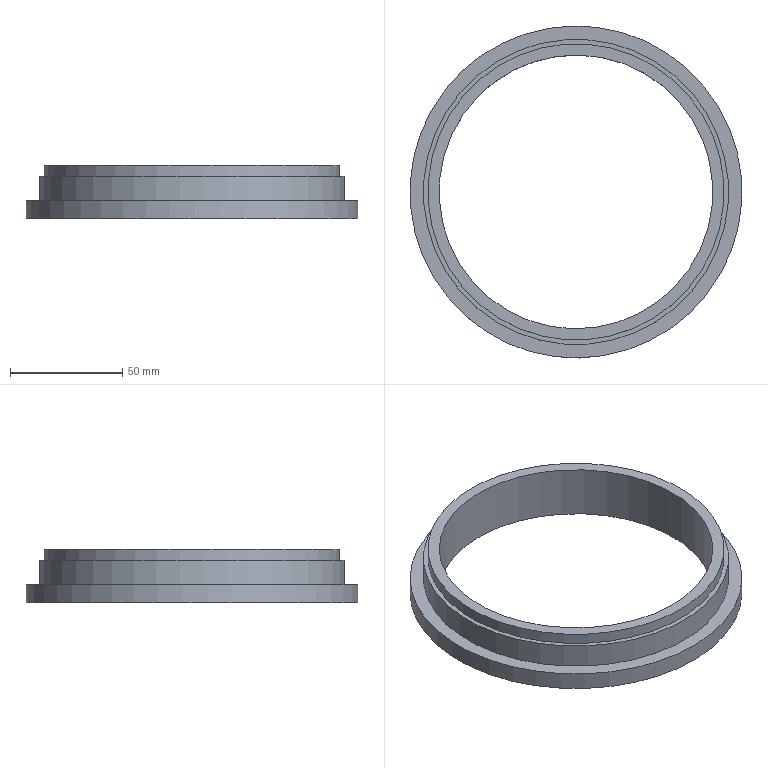Component | NX | CH3404-8 | 1 solid | 8 faces | box 148 x 148 x 24 mm | volume 85288 mm3 | cylinder 4 | plane 4 | commonest cylinder face diameters 122 x1 132 x1 136 x1 148 x1
STEP:
#1=CARTESIAN_POINT('',(0.,0.,0.));
#2=DIRECTION('',(0.,0.,1.));
#3=DIRECTION('',(1.,0.,0.));
#4=AXIS2_PLACEMENT_3D('',#1,#2,#3);
#5=CARTESIAN_POINT('',(56.878,23.472,-1551.3));
#6=VERTEX_POINT('',#5);
#7=CARTESIAN_POINT('',(0.5308,0.1057,-1551.3));
#8=DIRECTION('',(0.,0.,1.));
#9=DIRECTION('',(0.9237,0.383,0.));
#10=AXIS2_PLACEMENT_3D('',#7,#8,#9);
#11=CIRCLE('',#10,61.);
#12=CARTESIAN_POINT('',(0.5308,0.1057,-1551.3));
#13=DIRECTION('',(0.,0.,1.));
#14=DIRECTION('',(0.9237,0.383,0.));
#15=AXIS2_PLACEMENT_3D('',#12,#13,#14);
#16=CYLINDRICAL_SURFACE('',#15,61.);
#17=CARTESIAN_POINT('',(0.,0.));
#18=DIRECTION('',(1.,0.));
#19=VECTOR('',#18,1.);
#20=LINE('',#17,#19);
#21=(GEOMETRIC_REPRESENTATION_CONTEXT(2)PARAMETRIC_REPRESENTATION_CONTEXT()REPRESENTATION_CONTEXT('',''));
#22=DEFINITIONAL_REPRESENTATION('',(#20),#21);
#23=PCURVE('',#16,#22);
#24=CARTESIAN_POINT('',(-22.835,56.453,-1551.3));
#25=DIRECTION('',(0.,0.,1.));
#26=DIRECTION('',(0.9237,0.383,0.));
#27=AXIS2_PLACEMENT_3D('',#24,#25,#26);
#28=PLANE('',#27);
#29=CARTESIAN_POINT('',(-0.,-61.));
#30=DIRECTION('',(1.,0.));
#31=AXIS2_PLACEMENT_2D('',#29,#30);
#32=CIRCLE('',#31,61.);
#33=(GEOMETRIC_REPRESENTATION_CONTEXT(2)PARAMETRIC_REPRESENTATION_CONTEXT()REPRESENTATION_CONTEXT('',''));
#34=DEFINITIONAL_REPRESENTATION('',(#32),#33);
#35=PCURVE('',#28,#34);
#36=SURFACE_CURVE('',#11,(#23,#35),.PCURVE_S1.);
#37=EDGE_CURVE('',#6,#6,#36,.T.);
#38=ORIENTED_EDGE('',*,*,#37,.F.);
#39=CARTESIAN_POINT('',(56.878,23.472,-1575.3));
#40=VERTEX_POINT('',#39);
#41=CARTESIAN_POINT('',(56.878,23.472,-1575.3));
#42=CARTESIAN_POINT('',(56.878,23.472,-1551.3));
#43=B_SPLINE_CURVE_WITH_KNOTS('',1,(#41,#42),.UNSPECIFIED.,.F.,.F.,(2,2),(-24.,0.),.PIECEWISE_BEZIER_KNOTS.);
#44=CARTESIAN_POINT('',(0.,0.));
#45=DIRECTION('',(0.,1.));
#46=VECTOR('',#45,1.);
#47=LINE('',#44,#46);
#48=(GEOMETRIC_REPRESENTATION_CONTEXT(2)PARAMETRIC_REPRESENTATION_CONTEXT()REPRESENTATION_CONTEXT('',''));
#49=DEFINITIONAL_REPRESENTATION('',(#47),#48);
#50=PCURVE('',#16,#49);
#51=CARTESIAN_POINT('',(6.283,0.));
#52=DIRECTION('',(0.,1.));
#53=VECTOR('',#52,1.);
#54=LINE('',#51,#53);
#55=(GEOMETRIC_REPRESENTATION_CONTEXT(2)PARAMETRIC_REPRESENTATION_CONTEXT()REPRESENTATION_CONTEXT('',''));
#56=DEFINITIONAL_REPRESENTATION('',(#54),#55);
#57=PCURVE('',#16,#56);
#58=SEAM_CURVE('',#43,(#50,#57),.PCURVE_S1.);
#59=EDGE_CURVE('',#40,#6,#58,.T.);
#60=ORIENTED_EDGE('',*,*,#59,.F.);
#61=CARTESIAN_POINT('',(0.5308,0.1057,-1575.3));
#62=DIRECTION('',(0.,0.,1.));
#63=DIRECTION('',(0.9237,0.383,0.));
#64=AXIS2_PLACEMENT_3D('',#61,#62,#63);
#65=CIRCLE('',#64,61.);
#66=CARTESIAN_POINT('',(0.,-24.));
#67=DIRECTION('',(1.,0.));
#68=VECTOR('',#67,1.);
#69=LINE('',#66,#68);
#70=(GEOMETRIC_REPRESENTATION_CONTEXT(2)PARAMETRIC_REPRESENTATION_CONTEXT()REPRESENTATION_CONTEXT('',''));
#71=DEFINITIONAL_REPRESENTATION('',(#69),#70);
#72=PCURVE('',#16,#71);
#73=CARTESIAN_POINT('',(-27.815,68.462,-1575.3));
#74=DIRECTION('',(0.,0.,-1.));
#75=DIRECTION('',(-0.9237,-0.383,0.));
#76=AXIS2_PLACEMENT_3D('',#73,#74,#75);
#77=PLANE('',#76);
#78=CARTESIAN_POINT('',(-61.,-74.));
#79=CARTESIAN_POINT('',(-61.,31.655));
#80=CARTESIAN_POINT('',(30.5,-21.172));
#81=CARTESIAN_POINT('',(122.,-74.));
#82=CARTESIAN_POINT('',(30.5,-126.828));
#83=CARTESIAN_POINT('',(-61.,-179.655));
#84=CARTESIAN_POINT('',(-61.,-74.));
#85=(BOUNDED_CURVE()B_SPLINE_CURVE(2,(#78,#79,#80,#81,#82,#83,#84),.UNSPECIFIED.,.T.,.F.)B_SPLINE_CURVE_WITH_KNOTS((1,2,2,2,2,1),(-2.094,0.,2.094,4.189,6.283,8.378),.UNSPECIFIED.)CURVE()GEOMETRIC_REPRESENTATION_ITEM()RATIONAL_B_SPLINE_CURVE((1.,0.5,1.,0.5,1.,0.5,1.))REPRESENTATION_ITEM(''));
#86=(GEOMETRIC_REPRESENTATION_CONTEXT(2)PARAMETRIC_REPRESENTATION_CONTEXT()REPRESENTATION_CONTEXT('',''));
#87=DEFINITIONAL_REPRESENTATION('',(#85),#86);
#88=PCURVE('',#77,#87);
#89=SURFACE_CURVE('',#65,(#72,#88),.PCURVE_S1.);
#90=EDGE_CURVE('',#40,#40,#89,.T.);
#91=ORIENTED_EDGE('',*,*,#90,.T.);
#92=ORIENTED_EDGE('',*,*,#59,.T.);
#93=EDGE_LOOP('',(#38,#60,#91,#92));
#94=FACE_BOUND('',#93,.F.);
#95=ADVANCED_FACE('',(#94),#16,.F.);
#96=CARTESIAN_POINT('',(61.497,25.387,-1551.3));
#97=VERTEX_POINT('',#96);
#98=CARTESIAN_POINT('',(0.5308,0.1057,-1551.3));
#99=DIRECTION('',(0.,0.,1.));
#100=DIRECTION('',(0.9237,0.383,0.));
#101=AXIS2_PLACEMENT_3D('',#98,#99,#100);
#102=CIRCLE('',#101,66.);
#103=CARTESIAN_POINT('',(-0.,-61.));
#104=DIRECTION('',(1.,0.));
#105=AXIS2_PLACEMENT_2D('',#103,#104);
#106=CIRCLE('',#105,66.);
#107=(GEOMETRIC_REPRESENTATION_CONTEXT(2)PARAMETRIC_REPRESENTATION_CONTEXT()REPRESENTATION_CONTEXT('',''));
#108=DEFINITIONAL_REPRESENTATION('',(#106),#107);
#109=PCURVE('',#28,#108);
#110=CARTESIAN_POINT('',(0.5308,0.1057,-1551.3));
#111=DIRECTION('',(0.,0.,1.));
#112=DIRECTION('',(0.9237,0.383,0.));
#113=AXIS2_PLACEMENT_3D('',#110,#111,#112);
#114=CYLINDRICAL_SURFACE('',#113,66.);
#115=CARTESIAN_POINT('',(0.,0.));
#116=DIRECTION('',(1.,0.));
#117=VECTOR('',#116,1.);
#118=LINE('',#115,#117);
#119=(GEOMETRIC_REPRESENTATION_CONTEXT(2)PARAMETRIC_REPRESENTATION_CONTEXT()REPRESENTATION_CONTEXT('',''));
#120=DEFINITIONAL_REPRESENTATION('',(#118),#119);
#121=PCURVE('',#114,#120);
#122=SURFACE_CURVE('',#102,(#109,#121),.PCURVE_S1.);
#123=EDGE_CURVE('',#97,#97,#122,.T.);
#124=ORIENTED_EDGE('',*,*,#123,.T.);
#125=EDGE_LOOP('',(#124));
#126=FACE_BOUND('',#125,.T.);
#127=ORIENTED_EDGE('',*,*,#37,.F.);
#128=EDGE_LOOP('',(#127));
#129=FACE_BOUND('',#128,.T.);
#130=ADVANCED_FACE('',(#126,#129),#28,.T.);
#131=CARTESIAN_POINT('',(61.497,25.387,-1556.3));
#132=VERTEX_POINT('',#131);
#133=CARTESIAN_POINT('',(0.5308,0.1057,-1556.3));
#134=DIRECTION('',(0.,0.,1.));
#135=DIRECTION('',(0.9237,0.383,0.));
#136=AXIS2_PLACEMENT_3D('',#133,#134,#135);
#137=CIRCLE('',#136,66.);
#138=CARTESIAN_POINT('',(0.,-5.));
#139=DIRECTION('',(1.,0.));
#140=VECTOR('',#139,1.);
#141=LINE('',#138,#140);
#142=(GEOMETRIC_REPRESENTATION_CONTEXT(2)PARAMETRIC_REPRESENTATION_CONTEXT()REPRESENTATION_CONTEXT('',''));
#143=DEFINITIONAL_REPRESENTATION('',(#141),#142);
#144=PCURVE('',#114,#143);
#145=CARTESIAN_POINT('',(-24.75,61.072,-1556.3));
#146=DIRECTION('',(0.,0.,1.));
#147=DIRECTION('',(0.9237,0.383,0.));
#148=AXIS2_PLACEMENT_3D('',#145,#146,#147);
#149=PLANE('',#148);
#150=CARTESIAN_POINT('',(-0.,-66.));
#151=DIRECTION('',(1.,0.));
#152=AXIS2_PLACEMENT_2D('',#150,#151);
#153=CIRCLE('',#152,66.);
#154=(GEOMETRIC_REPRESENTATION_CONTEXT(2)PARAMETRIC_REPRESENTATION_CONTEXT()REPRESENTATION_CONTEXT('',''));
#155=DEFINITIONAL_REPRESENTATION('',(#153),#154);
#156=PCURVE('',#149,#155);
#157=SURFACE_CURVE('',#137,(#144,#156),.PCURVE_S1.);
#158=EDGE_CURVE('',#132,#132,#157,.T.);
#159=ORIENTED_EDGE('',*,*,#158,.T.);
#160=CARTESIAN_POINT('',(61.497,25.387,-1556.3));
#161=CARTESIAN_POINT('',(61.497,25.387,-1551.3));
#162=B_SPLINE_CURVE_WITH_KNOTS('',1,(#160,#161),.UNSPECIFIED.,.F.,.F.,(2,2),(-5.,0.),.PIECEWISE_BEZIER_KNOTS.);
#163=CARTESIAN_POINT('',(6.283,0.));
#164=DIRECTION('',(0.,1.));
#165=VECTOR('',#164,1.);
#166=LINE('',#163,#165);
#167=(GEOMETRIC_REPRESENTATION_CONTEXT(2)PARAMETRIC_REPRESENTATION_CONTEXT()REPRESENTATION_CONTEXT('',''));
#168=DEFINITIONAL_REPRESENTATION('',(#166),#167);
#169=PCURVE('',#114,#168);
#170=CARTESIAN_POINT('',(0.,0.));
#171=DIRECTION('',(0.,1.));
#172=VECTOR('',#171,1.);
#173=LINE('',#170,#172);
#174=(GEOMETRIC_REPRESENTATION_CONTEXT(2)PARAMETRIC_REPRESENTATION_CONTEXT()REPRESENTATION_CONTEXT('',''));
#175=DEFINITIONAL_REPRESENTATION('',(#173),#174);
#176=PCURVE('',#114,#175);
#177=SEAM_CURVE('',#162,(#169,#176),.PCURVE_S1.);
#178=EDGE_CURVE('',#132,#97,#177,.T.);
#179=ORIENTED_EDGE('',*,*,#178,.T.);
#180=ORIENTED_EDGE('',*,*,#123,.F.);
#181=ORIENTED_EDGE('',*,*,#178,.F.);
#182=EDGE_LOOP('',(#159,#179,#180,#181));
#183=FACE_BOUND('',#182,.T.);
#184=ADVANCED_FACE('',(#183),#114,.T.);
#185=CARTESIAN_POINT('',(63.344,26.153,-1556.3));
#186=VERTEX_POINT('',#185);
#187=CARTESIAN_POINT('',(0.5308,0.1057,-1556.3));
#188=DIRECTION('',(0.,0.,1.));
#189=DIRECTION('',(0.9237,0.383,0.));
#190=AXIS2_PLACEMENT_3D('',#187,#188,#189);
#191=CIRCLE('',#190,68.);
#192=CARTESIAN_POINT('',(-0.,-66.));
#193=DIRECTION('',(1.,0.));
#194=AXIS2_PLACEMENT_2D('',#192,#193);
#195=CIRCLE('',#194,68.);
#196=(GEOMETRIC_REPRESENTATION_CONTEXT(2)PARAMETRIC_REPRESENTATION_CONTEXT()REPRESENTATION_CONTEXT('',''));
#197=DEFINITIONAL_REPRESENTATION('',(#195),#196);
#198=PCURVE('',#149,#197);
#199=CARTESIAN_POINT('',(0.5308,0.1057,-1551.3));
#200=DIRECTION('',(0.,0.,1.));
#201=DIRECTION('',(0.9237,0.383,0.));
#202=AXIS2_PLACEMENT_3D('',#199,#200,#201);
#203=CYLINDRICAL_SURFACE('',#202,68.);
#204=CARTESIAN_POINT('',(0.,-5.));
#205=DIRECTION('',(1.,0.));
#206=VECTOR('',#205,1.);
#207=LINE('',#204,#206);
#208=(GEOMETRIC_REPRESENTATION_CONTEXT(2)PARAMETRIC_REPRESENTATION_CONTEXT()REPRESENTATION_CONTEXT('',''));
#209=DEFINITIONAL_REPRESENTATION('',(#207),#208);
#210=PCURVE('',#203,#209);
#211=SURFACE_CURVE('',#191,(#198,#210),.PCURVE_S1.);
#212=EDGE_CURVE('',#186,#186,#211,.T.);
#213=ORIENTED_EDGE('',*,*,#212,.T.);
#214=EDGE_LOOP('',(#213));
#215=FACE_BOUND('',#214,.T.);
#216=ORIENTED_EDGE('',*,*,#158,.F.);
#217=EDGE_LOOP('',(#216));
#218=FACE_BOUND('',#217,.T.);
#219=ADVANCED_FACE('',(#215,#218),#149,.T.);
#220=CARTESIAN_POINT('',(63.344,26.153,-1567.3));
#221=VERTEX_POINT('',#220);
#222=CARTESIAN_POINT('',(0.5308,0.1057,-1567.3));
#223=DIRECTION('',(0.,0.,1.));
#224=DIRECTION('',(0.9237,0.383,0.));
#225=AXIS2_PLACEMENT_3D('',#222,#223,#224);
#226=CIRCLE('',#225,68.);
#227=CARTESIAN_POINT('',(0.,-16.));
#228=DIRECTION('',(1.,0.));
#229=VECTOR('',#228,1.);
#230=LINE('',#227,#229);
#231=(GEOMETRIC_REPRESENTATION_CONTEXT(2)PARAMETRIC_REPRESENTATION_CONTEXT()REPRESENTATION_CONTEXT('',''));
#232=DEFINITIONAL_REPRESENTATION('',(#230),#231);
#233=PCURVE('',#203,#232);
#234=CARTESIAN_POINT('',(-25.517,62.919,-1567.3));
#235=DIRECTION('',(0.,0.,1.));
#236=DIRECTION('',(0.9237,0.383,0.));
#237=AXIS2_PLACEMENT_3D('',#234,#235,#236);
#238=PLANE('',#237);
#239=CARTESIAN_POINT('',(-0.,-68.));
#240=DIRECTION('',(1.,0.));
#241=AXIS2_PLACEMENT_2D('',#239,#240);
#242=CIRCLE('',#241,68.);
#243=(GEOMETRIC_REPRESENTATION_CONTEXT(2)PARAMETRIC_REPRESENTATION_CONTEXT()REPRESENTATION_CONTEXT('',''));
#244=DEFINITIONAL_REPRESENTATION('',(#242),#243);
#245=PCURVE('',#238,#244);
#246=SURFACE_CURVE('',#226,(#233,#245),.PCURVE_S1.);
#247=EDGE_CURVE('',#221,#221,#246,.T.);
#248=ORIENTED_EDGE('',*,*,#247,.T.);
#249=CARTESIAN_POINT('',(63.344,26.153,-1567.3));
#250=CARTESIAN_POINT('',(63.344,26.153,-1556.3));
#251=B_SPLINE_CURVE_WITH_KNOTS('',1,(#249,#250),.UNSPECIFIED.,.F.,.F.,(2,2),(-16.,-5.),.PIECEWISE_BEZIER_KNOTS.);
#252=CARTESIAN_POINT('',(6.283,0.));
#253=DIRECTION('',(0.,1.));
#254=VECTOR('',#253,1.);
#255=LINE('',#252,#254);
#256=(GEOMETRIC_REPRESENTATION_CONTEXT(2)PARAMETRIC_REPRESENTATION_CONTEXT()REPRESENTATION_CONTEXT('',''));
#257=DEFINITIONAL_REPRESENTATION('',(#255),#256);
#258=PCURVE('',#203,#257);
#259=CARTESIAN_POINT('',(0.,0.));
#260=DIRECTION('',(0.,1.));
#261=VECTOR('',#260,1.);
#262=LINE('',#259,#261);
#263=(GEOMETRIC_REPRESENTATION_CONTEXT(2)PARAMETRIC_REPRESENTATION_CONTEXT()REPRESENTATION_CONTEXT('',''));
#264=DEFINITIONAL_REPRESENTATION('',(#262),#263);
#265=PCURVE('',#203,#264);
#266=SEAM_CURVE('',#251,(#258,#265),.PCURVE_S1.);
#267=EDGE_CURVE('',#221,#186,#266,.T.);
#268=ORIENTED_EDGE('',*,*,#267,.T.);
#269=ORIENTED_EDGE('',*,*,#212,.F.);
#270=ORIENTED_EDGE('',*,*,#267,.F.);
#271=EDGE_LOOP('',(#248,#268,#269,#270));
#272=FACE_BOUND('',#271,.T.);
#273=ADVANCED_FACE('',(#272),#203,.T.);
#274=CARTESIAN_POINT('',(68.887,28.451,-1567.3));
#275=VERTEX_POINT('',#274);
#276=CARTESIAN_POINT('',(0.5308,0.1057,-1567.3));
#277=DIRECTION('',(0.,0.,1.));
#278=DIRECTION('',(0.9237,0.383,0.));
#279=AXIS2_PLACEMENT_3D('',#276,#277,#278);
#280=CIRCLE('',#279,74.);
#281=CARTESIAN_POINT('',(-0.,-68.));
#282=DIRECTION('',(1.,0.));
#283=AXIS2_PLACEMENT_2D('',#281,#282);
#284=CIRCLE('',#283,74.);
#285=(GEOMETRIC_REPRESENTATION_CONTEXT(2)PARAMETRIC_REPRESENTATION_CONTEXT()REPRESENTATION_CONTEXT('',''));
#286=DEFINITIONAL_REPRESENTATION('',(#284),#285);
#287=PCURVE('',#238,#286);
#288=CARTESIAN_POINT('',(0.5308,0.1057,-1551.3));
#289=DIRECTION('',(0.,0.,1.));
#290=DIRECTION('',(0.9237,0.383,0.));
#291=AXIS2_PLACEMENT_3D('',#288,#289,#290);
#292=CYLINDRICAL_SURFACE('',#291,74.);
#293=CARTESIAN_POINT('',(0.,-16.));
#294=DIRECTION('',(1.,0.));
#295=VECTOR('',#294,1.);
#296=LINE('',#293,#295);
#297=(GEOMETRIC_REPRESENTATION_CONTEXT(2)PARAMETRIC_REPRESENTATION_CONTEXT()REPRESENTATION_CONTEXT('',''));
#298=DEFINITIONAL_REPRESENTATION('',(#296),#297);
#299=PCURVE('',#292,#298);
#300=SURFACE_CURVE('',#280,(#287,#299),.PCURVE_S1.);
#301=EDGE_CURVE('',#275,#275,#300,.T.);
#302=ORIENTED_EDGE('',*,*,#301,.T.);
#303=EDGE_LOOP('',(#302));
#304=FACE_BOUND('',#303,.T.);
#305=ORIENTED_EDGE('',*,*,#247,.F.);
#306=EDGE_LOOP('',(#305));
#307=FACE_BOUND('',#306,.T.);
#308=ADVANCED_FACE('',(#304,#307),#238,.T.);
#309=CARTESIAN_POINT('',(68.887,28.451,-1575.3));
#310=VERTEX_POINT('',#309);
#311=CARTESIAN_POINT('',(0.5308,0.1057,-1575.3));
#312=DIRECTION('',(0.,0.,1.));
#313=DIRECTION('',(0.9237,0.383,0.));
#314=AXIS2_PLACEMENT_3D('',#311,#312,#313);
#315=CIRCLE('',#314,74.);
#316=CARTESIAN_POINT('',(0.,-24.));
#317=DIRECTION('',(1.,0.));
#318=VECTOR('',#317,1.);
#319=LINE('',#316,#318);
#320=(GEOMETRIC_REPRESENTATION_CONTEXT(2)PARAMETRIC_REPRESENTATION_CONTEXT()REPRESENTATION_CONTEXT('',''));
#321=DEFINITIONAL_REPRESENTATION('',(#319),#320);
#322=PCURVE('',#292,#321);
#323=CARTESIAN_POINT('',(-74.,-74.));
#324=CARTESIAN_POINT('',(-74.,54.172));
#325=CARTESIAN_POINT('',(37.,-9.914));
#326=CARTESIAN_POINT('',(148.,-74.));
#327=CARTESIAN_POINT('',(37.,-138.086));
#328=CARTESIAN_POINT('',(-74.,-202.172));
#329=CARTESIAN_POINT('',(-74.,-74.));
#330=(BOUNDED_CURVE()B_SPLINE_CURVE(2,(#323,#324,#325,#326,#327,#328,#329),.UNSPECIFIED.,.T.,.F.)B_SPLINE_CURVE_WITH_KNOTS((1,2,2,2,2,1),(-2.094,0.,2.094,4.189,6.283,8.378),.UNSPECIFIED.)CURVE()GEOMETRIC_REPRESENTATION_ITEM()RATIONAL_B_SPLINE_CURVE((1.,0.5,1.,0.5,1.,0.5,1.))REPRESENTATION_ITEM(''));
#331=(GEOMETRIC_REPRESENTATION_CONTEXT(2)PARAMETRIC_REPRESENTATION_CONTEXT()REPRESENTATION_CONTEXT('',''));
#332=DEFINITIONAL_REPRESENTATION('',(#330),#331);
#333=PCURVE('',#77,#332);
#334=SURFACE_CURVE('',#315,(#322,#333),.PCURVE_S1.);
#335=EDGE_CURVE('',#310,#310,#334,.T.);
#336=ORIENTED_EDGE('',*,*,#335,.T.);
#337=CARTESIAN_POINT('',(68.887,28.451,-1575.3));
#338=CARTESIAN_POINT('',(68.887,28.451,-1567.3));
#339=B_SPLINE_CURVE_WITH_KNOTS('',1,(#337,#338),.UNSPECIFIED.,.F.,.F.,(2,2),(-24.,-16.),.PIECEWISE_BEZIER_KNOTS.);
#340=CARTESIAN_POINT('',(6.283,0.));
#341=DIRECTION('',(0.,1.));
#342=VECTOR('',#341,1.);
#343=LINE('',#340,#342);
#344=(GEOMETRIC_REPRESENTATION_CONTEXT(2)PARAMETRIC_REPRESENTATION_CONTEXT()REPRESENTATION_CONTEXT('',''));
#345=DEFINITIONAL_REPRESENTATION('',(#343),#344);
#346=PCURVE('',#292,#345);
#347=CARTESIAN_POINT('',(0.,0.));
#348=DIRECTION('',(0.,1.));
#349=VECTOR('',#348,1.);
#350=LINE('',#347,#349);
#351=(GEOMETRIC_REPRESENTATION_CONTEXT(2)PARAMETRIC_REPRESENTATION_CONTEXT()REPRESENTATION_CONTEXT('',''));
#352=DEFINITIONAL_REPRESENTATION('',(#350),#351);
#353=PCURVE('',#292,#352);
#354=SEAM_CURVE('',#339,(#346,#353),.PCURVE_S1.);
#355=EDGE_CURVE('',#310,#275,#354,.T.);
#356=ORIENTED_EDGE('',*,*,#355,.T.);
#357=ORIENTED_EDGE('',*,*,#301,.F.);
#358=ORIENTED_EDGE('',*,*,#355,.F.);
#359=EDGE_LOOP('',(#336,#356,#357,#358));
#360=FACE_BOUND('',#359,.T.);
#361=ADVANCED_FACE('',(#360),#292,.T.);
#362=ORIENTED_EDGE('',*,*,#90,.T.);
#363=EDGE_LOOP('',(#362));
#364=FACE_BOUND('',#363,.T.);
#365=ORIENTED_EDGE('',*,*,#335,.F.);
#366=EDGE_LOOP('',(#365));
#367=FACE_BOUND('',#366,.T.);
#368=ADVANCED_FACE('',(#364,#367),#77,.T.);
#369=CLOSED_SHELL('',(#95,#130,#184,#219,#273,#308,#361,#368));
#370=MANIFOLD_SOLID_BREP('',#369);
#371=(LENGTH_UNIT()NAMED_UNIT(*)SI_UNIT(.MILLI.,.METRE.));
#372=UNCERTAINTY_MEASURE_WITH_UNIT(LENGTH_MEASURE(0.00001),#371,'','');
#373=(NAMED_UNIT(*)PLANE_ANGLE_UNIT()SI_UNIT($,.RADIAN.));
#374=(NAMED_UNIT(*)SI_UNIT($,.STERADIAN.)SOLID_ANGLE_UNIT());
#375=(GEOMETRIC_REPRESENTATION_CONTEXT(3)GLOBAL_UNCERTAINTY_ASSIGNED_CONTEXT((#372))GLOBAL_UNIT_ASSIGNED_CONTEXT((#371,#373,#374))REPRESENTATION_CONTEXT('',''));
#376=ADVANCED_BREP_SHAPE_REPRESENTATION('',(#4,#370),#375);